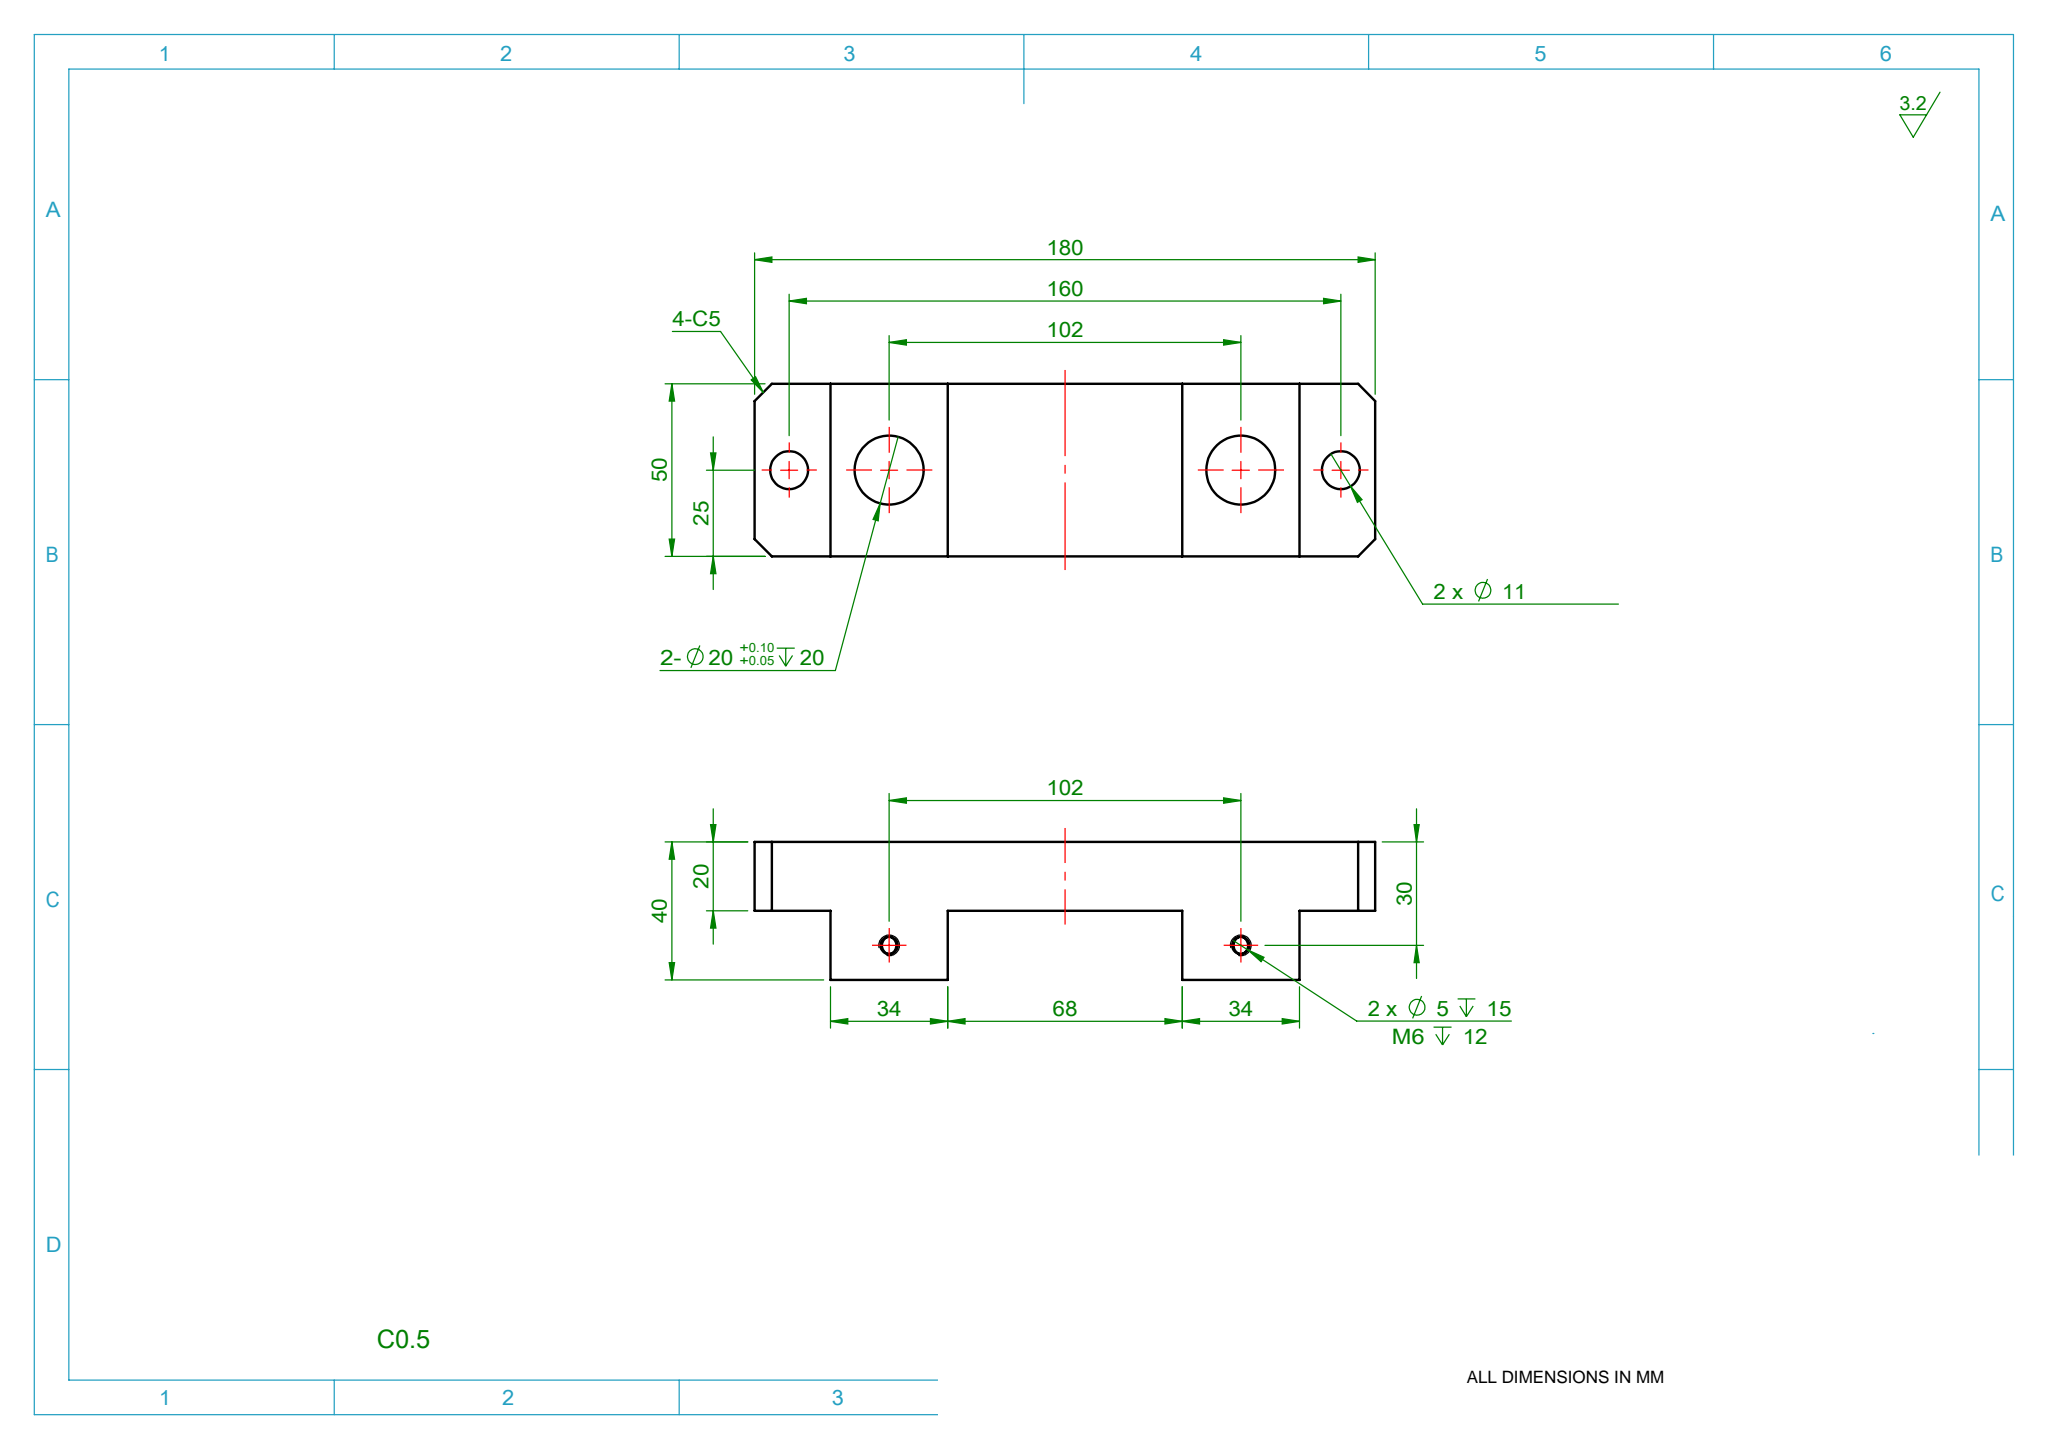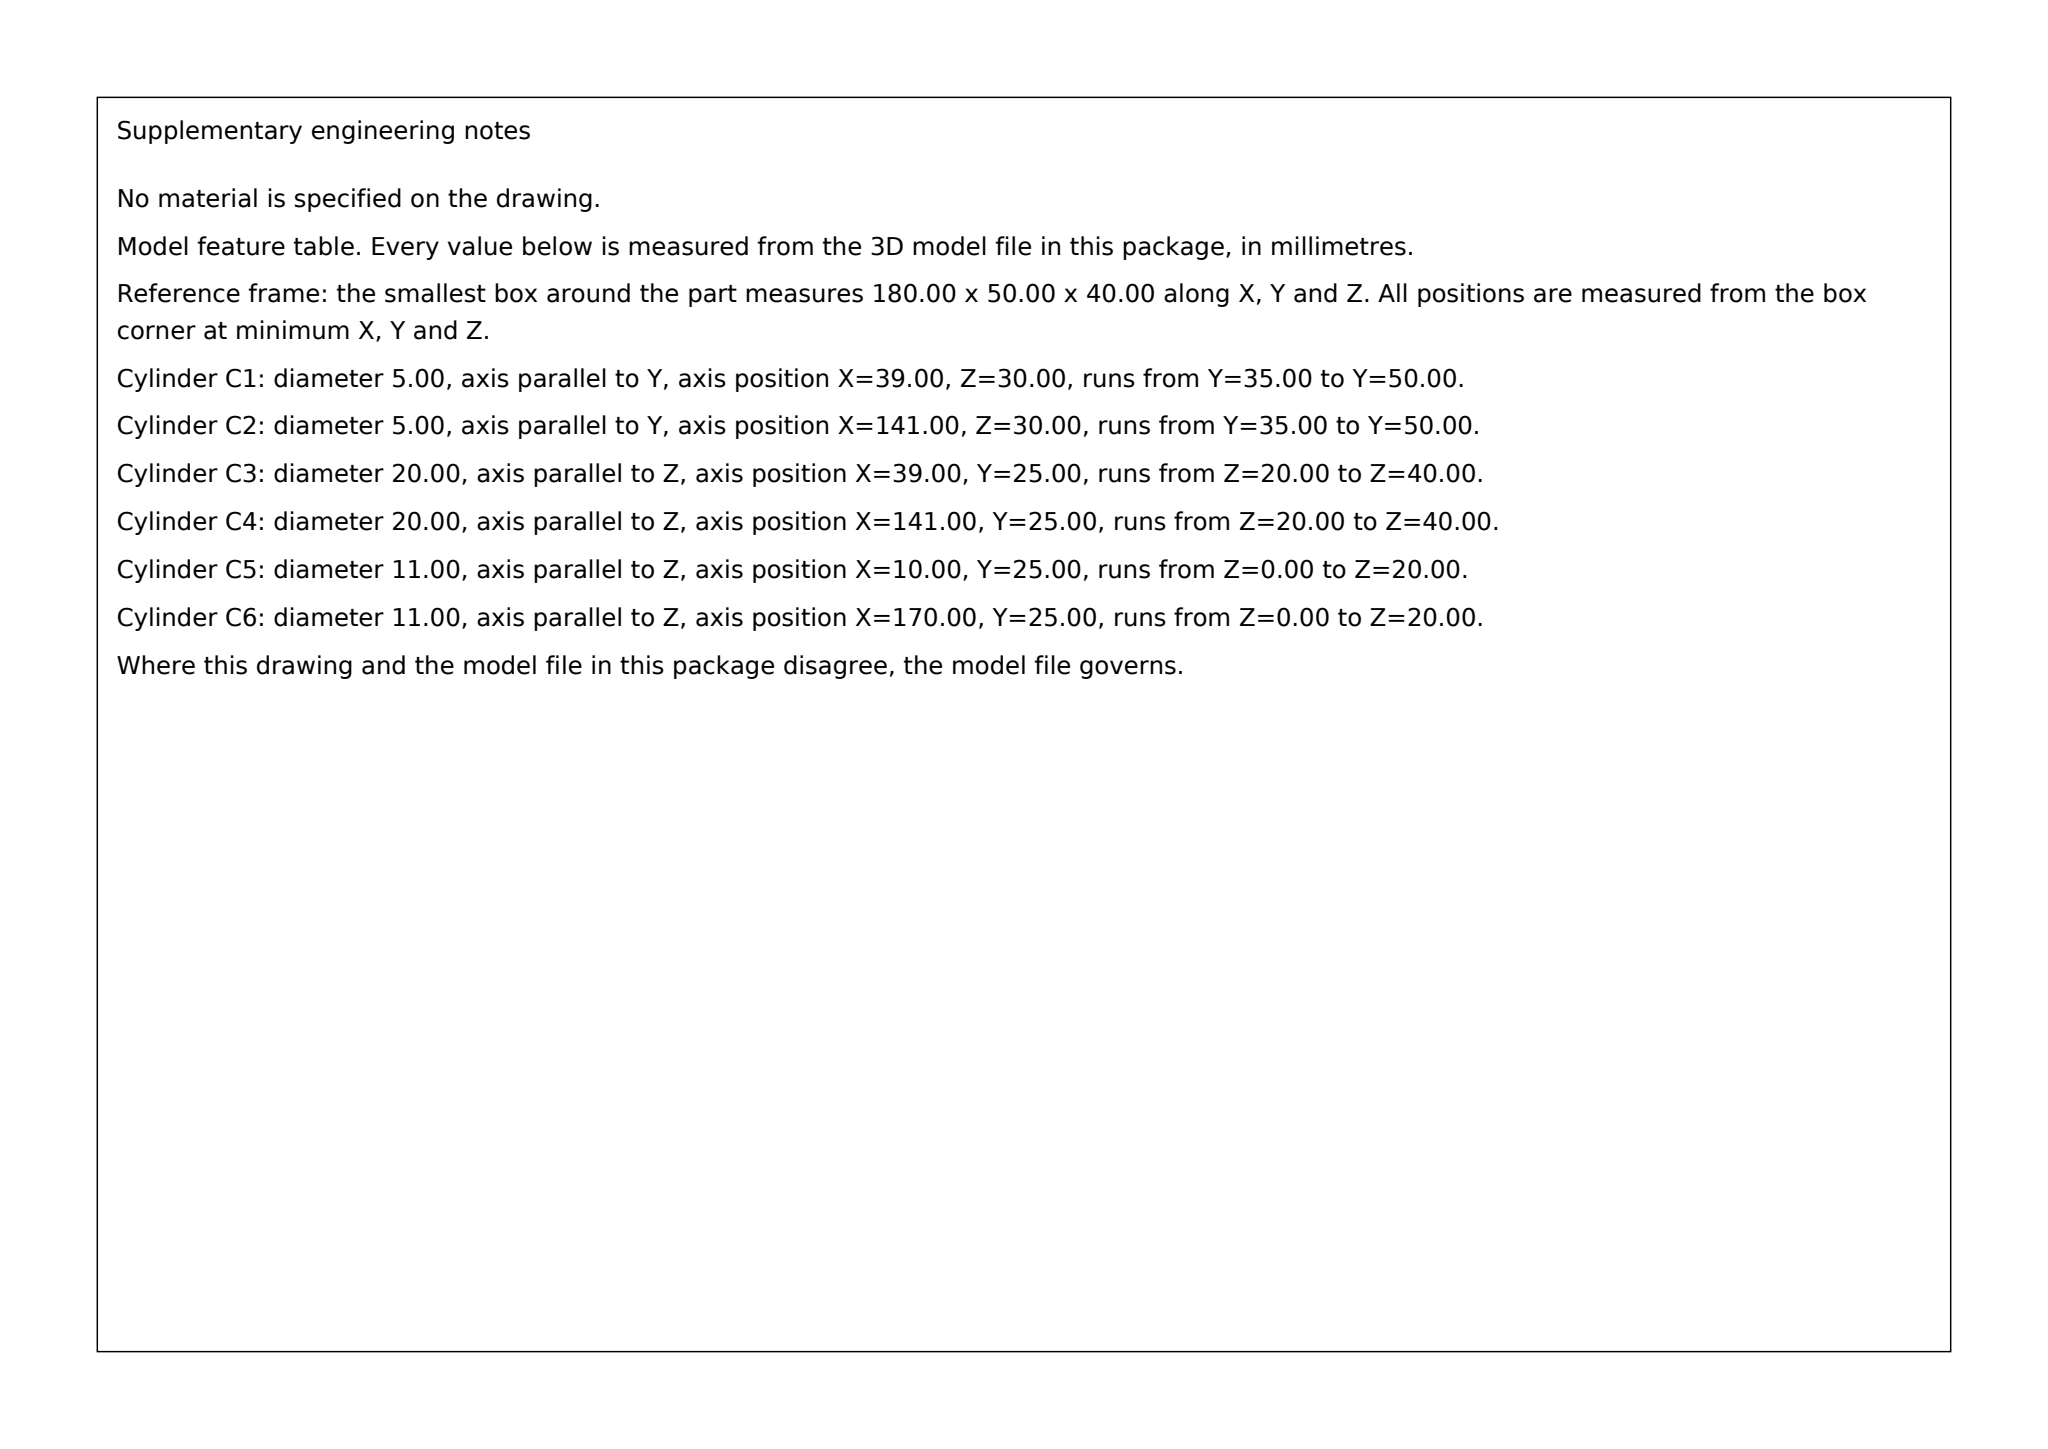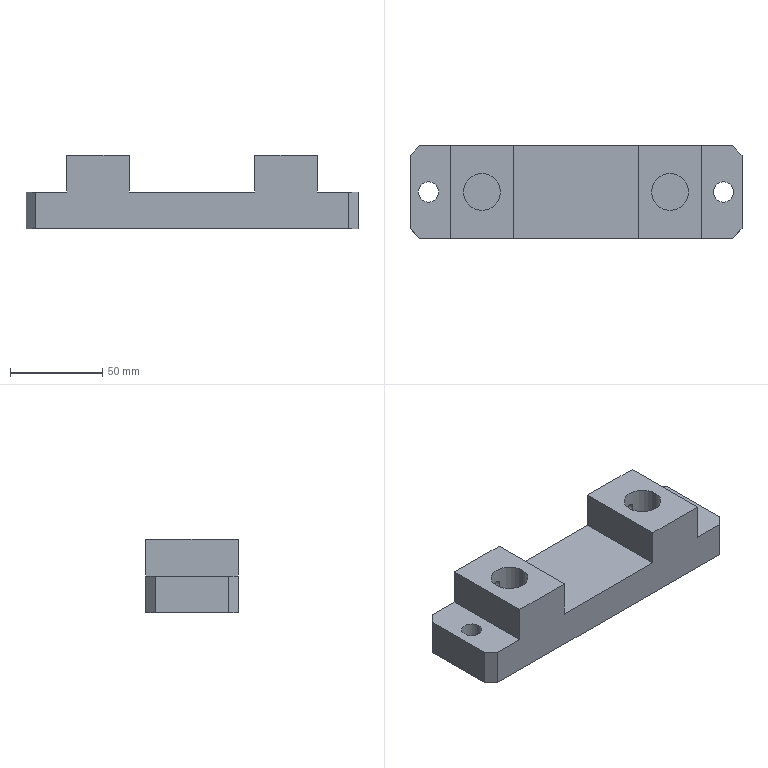Part | SolidWorks | mm | 1 solid | 36 faces | box 180 x 50 x 40 mm | volume 230041 mm3 | plane 20 | cylinder 12 | cone 4 | commonest cylinder face diameters 5 x4 11 x4 20 x4
build123d program:
from build123d import *

# Parameters (mm, degrees)
BOSS_EXTRUDE1_DEPTH   = 50
SKETCH2_R             = 10
CUT_EXTRUDE1_DEPTH    = 20
M10_CLEARANCE_HOLE1_D = 11
M6_TAPPED_HOLE1_D     = 5
M6_TAPPED_HOLE1_DEPTH = 15
M6_TAPPED_HOLE1_TIP   = 1.502
CHAMFER1_SIZE         = 5


with BuildPart() as part:
    # Sketch1 → Boss-Extrude1 (new body)
    with BuildSketch(Plane(origin=(0, 0, 0), x_dir=(1, 0, 0), z_dir=(0, 1, 0))):
        Polygon((0, 0), (180, 0), (180, -20), (158, -20), (158, -40), (124, -40), (124, -20), (56, -20), (56, -40), (22, -40), (22, -20), (0, -20), align=None)
    extrude(amount=BOSS_EXTRUDE1_DEPTH)

    # Sketch2 → Cut-Extrude1 (cut)
    with BuildSketch(Plane.XY.offset(40)):
        with Locations((39, 25)):
            Circle(SKETCH2_R)
        with Locations((141, 25)):
            Circle(SKETCH2_R)
    extrude(amount=-CUT_EXTRUDE1_DEPTH, mode=Mode.SUBTRACT)

    # M10 Clearance Hole1 (through all)
    with Locations(Plane.XY.offset(20)):
        with Locations((10, 25), (170, 25)):
            Hole(M10_CLEARANCE_HOLE1_D / 2)

    # M6 Tapped Hole1
    with Locations(Plane(origin=(0, 50, 0), x_dir=(1, 0, 0), z_dir=(0, 1, 0))):
        with Locations((39, -30), (141, -30)):
            Hole(M6_TAPPED_HOLE1_D / 2, depth=M6_TAPPED_HOLE1_DEPTH)
            with Locations((0, 0, -(M6_TAPPED_HOLE1_DEPTH + M6_TAPPED_HOLE1_TIP / 2))):  # 118° drill point
                Cone(0, M6_TAPPED_HOLE1_D / 2, M6_TAPPED_HOLE1_TIP, mode=Mode.SUBTRACT)

    # Chamfer1
    chamfer1_edges = [part.edges().sort_by_distance(p)[0] for p in [
        (180, 0, 10),
        (0, 0, 10),
        (180, 50, 10),
        (0, 50, 10),
    ]]
    chamfer(chamfer1_edges, length=CHAMFER1_SIZE)


solid = part.part